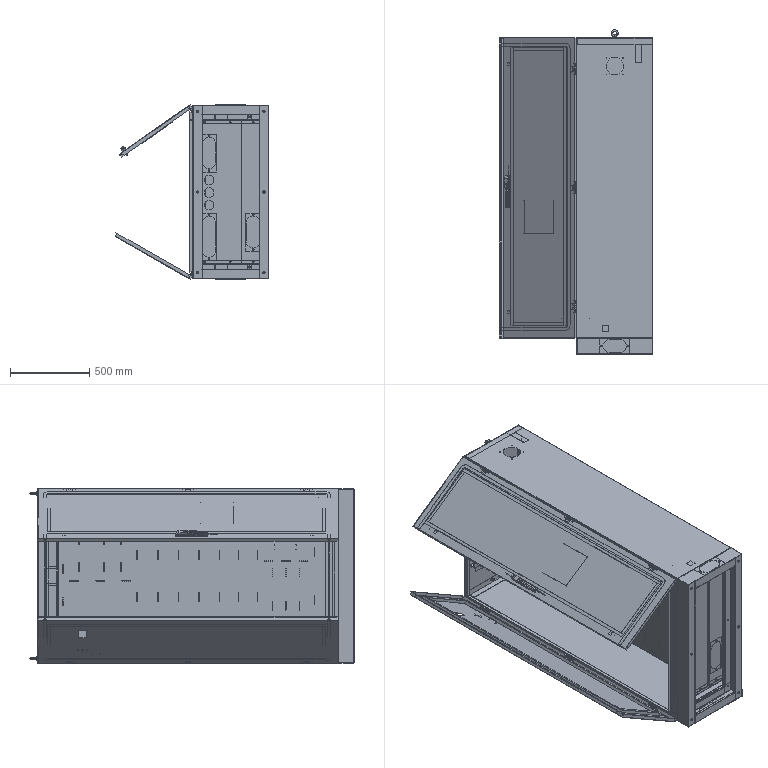Assembly | SolidWorks | mm | 69 component files | 71 solids | 3708 faces | box 971.82 x 2050.25 x 1105.32 mm | volume 17695028 mm3 | cylinder 1882 | plane 1722 | spline 100 | cone 4 | commonest cylinder face diameters 5 x728 7 x132 0.5 x108 0.2 x99 6 x92 3 x90 4 x86 8 x80
Bill of materials:
201LargeHinge | 6 |  | Elongated bracket with a hollow, open-sided box-section beam along one edge and a teardrop-profile side web ending in a cylindrical knuckle with a through bore; two knuckle segments are separated by a central gap, and internal cylindrical bosses with holes sit inside the beam.
BaseCableHoleBlankingPlate | 4 |  | Thin flat rectangular plate with two small round holes centered near its two short ends.
BottomFrameFront | 1 |  | Long, slender sheet-metal channel with a C-shaped cross-section, small-radius bends and short inward return lips; small holes are spaced along the length.
BottomFrameLeftAndRight | 2 |  | Sheet-metal cover/plate with a flat top panel, two bent-down side walls ending in short inward feet, flat end tabs extending past the walls, and a central obround cutout flanked by two small holes.
BottomFrameRear | 1 |  | Long sheet-metal channel with a C-shaped cross-section and short return lips; the web has two obround cutouts, each with small holes above and below it, plus small holes along the flanges and a small internal boss.
BottomBlankingPlateCableHoleBlankingPlate1 | 1 |  | Thin flat rectangular plate, narrower than tall, with two small round holes on the centerline near the short ends.
BottomBlankingPlateCableHoleBlankingPlate2 | 2 |  | Thin flat rectangular plate with two small round holes on the centerline near each short end.
BottomPlateMountingPlate1 | 1 |  | Flat rectangular sheet panel with very short bent edge flanges on the long sides; it has two large obround cutouts, three circular holes between them, small holes beside each cutout and small holes near the corners.
BottomPlateMountingPlate2 | 1 |  | Long, narrow flat sheet panel with short bent side flanges, a single obround cutout in the lower portion with small holes above and below it, and small holes near both ends.
ConnectingAngleIron | 1 |  | Thin L-shaped angle with roughly equal legs and a small inside bend radius; one leg is shorter in length than the other, which creates a step at one end.
ConnectingAngleIronSymmetric | 1 |  | Thin L-shaped angle with a small bend radius; the two legs differ in length, giving a step at one end. It appears to be a mirrored or reoriented version of a similar angle.
FrontLowerBeam | 1 |  | Long, slender sheet-metal profile with an asymmetric section: a top flange extending one way, a tall web, a bottom flange extending the other way and a short upturned lip; small holes are spaced along its length.
LeftSidePanel | 1 |  | Long, shallow rectangular tray made of thin plate. It has a flat base, low upturned flanges along both long edges and short turned-down end lips.
LimitSwitchBracket | 1 |  | Short equal-leg angle bracket with a rounded inside bend and two round through-holes in one leg.
MountingBeam | 1 |  | Long, slender angle profile with a rounded bend and one small hole near each end of one leg.
MountingPlateBracket | 2 |  | Square-legged L-bracket of thin plate with a round hole in the upright leg and a short cylindrical boss or sleeve on that leg.
RearDoorFixingPlate | 2 |  | Flat rectangular plate with two rounded corners along one edge and a large central round through-hole, similar to a square washer or tab.
RearLowerBeam | 1 |  | Long thin-walled formed profile with several bends, in a stepped open-channel shape. It has one small hole near mid-length and stepped or notched ends.
RightSidePlate | 1 |  | Long rectangular panel or cover with turned-down edges, one large round hole near one end and small holes around that hole.
ShelfSupportBeamLeft | 1 |  | Long stepped bracket rail with a Z- or hat-like section. It carries three evenly spaced cylindrical studs or bosses on one flange and a block-and-cylinder feature on another web.
ShelfSupportBeamRight | 1 |  | Long stepped bracket rail with a multi-bend profile, mirrored compared with unnamed part. It has three evenly spaced cylindrical studs or bosses.
TopCover | 1 |  | Rectangular sheet panel with stepped or offset flanges along its long edges. It has an obround slot near one end, small holes on either side of the slot, and small holes at the end centrelines.
TopLightBracket | 1 |  | Long C-channel with a flat web, short return flanges at each end of the section and two small holes in the web.
TopReinforcementAngleIron | 2 |  | Long equal-leg angle with one round hole at mid-length in the upright leg and a hex-shaped boss, likely a nut-like feature, on the inside face at that hole.
Triangle | 2 |  | Thin flat plate in the shape of a right triangle, with one circular through-hole near the right-angle corner.
CL201-1Hinge(ClawTypeAttachment) | 6 |  | Flat rectangular sheet leaf with one edge rolled into a hollow cylindrical barrel. The barrel is split into three knuckle segments separated by two gaps. It looks like a hinge leaf.
FrontDoorFlange | 1 |  | Long rectangular thin sheet panel with shallow turned-up or bent edges along the long sides and small notches near the ends. Near one end it has one small rectangular cutout and one small hole with small marks around it.
1760RectangularTube | 4 |  | Thin square frame made of slender bar stock with an open center. It looks like a closed square loop.
390RectangularTube | 4 |  | Straight bar with a square cross-section and flat square ends.
WireRack | 1 |  | Bent sheet strap: a flat rectangular web with a short leg bent down about 90 degrees at each end, forming a shallow U or cap profile with rounded bends.
DocumentBox | 1 |  | Rectangular flat plate or block with a V-shaped notch cut in from one edge. The notch ends in a rounded root.
FrontDoorLockHole | 1 |  | Long thin rectangular sheet panel with narrow bent edges along the long sides, small notches near the ends, and a few small slots or holes near one long edge.
LockRodBracket | 2 |  | L-shaped bent sheet bracket. One leg is a flat rectangle. The other leg, bent about 90 degrees, has a rounded end and a large circular through-hole.
LowerLockRod | 1 |  | Long slender round rod with a short jog (double bend) near one end and a pointed or chamfered tip at that end. The other end is a flattened section with two small holes.
M12LiftingEye | 2 |  | Eye-bolt-like part: a round ring (torus) joined to a cylindrical collar, with a smaller-diameter cylindrical shank extending from the collar.
MountingPlate | 1 |  | Long narrow sheet channel with a shallow U cross-section and rounded corners. There is one small elongated hole near each end of the web.
MS830ConnectingRodLock | 1 |  | Long, narrow multi-piece-looking body: a stepped, box-like housing with a chamfered upper end, sitting on a flat strip. The strip runs past both ends as flat tabs, each with two round holes, and is joggled (offset) where it leaves the housing. A small round knob or disc with a slot sits on one side face, near a rectangular block.
RearDoorPanel | 1 |  | Thin, flat rectangular plate, about twice as long as it is tall, with uniform thickness and no clear cutouts.
RearDoorStiffener | 1 |  | Long, straight, thin-walled formed profile of constant cross-section. The end view shows a hat (top-hat) shape: a central web, two legs turning toward the same side, and short lips at the ends of the legs turning away from each other.
Shelf | 1 |  | Thin, flat rectangular plate with many small perforations in short straight rows, mostly vertical with some horizontal, spread across the face in a grid-like layout.
TopCoverCableHoleBlankingPlate | 1 |  | Thin, flat rectangular plate, about twice as long as it is tall, with one round through-hole near each short end, both at mid-height.
UpperLockRod | 1 |  | Long, slender round rod. Near one end it has a short joggle (an offset bend in two steps), ending in a short straight tip. The other end is a short flattened or rectangular section with two small holes.
Mates:
1. coincident | CabinetWelding-1/FrontLowerBeam-1 face at (108.182, -1006.927, 1410.006) dir (0, -1, 0) | BaseWeldment-1/BottomFrameLeftAndRight-1 face at (-18040.001, -1006.927, 9206.843) dir (0, 1, 0)
2. coincident | CabinetWelding-1/RightSidePlate-1 face at (-10032.487, -6118.242, 2450.006) dir (0, 0, 1) | BaseWeldment-1/BottomFrameLeftAndRight-1 face at (-18040.001, -7766.065, 2450.006) dir (0, 0, 1)
3. coincident | CabinetWelding-1/FrontLowerBeam-1 face at (107.082, -1006.227, 1410.006) dir (-1, 0, 0) | BaseWeldment-1/BottomFrameFront-1 face at (107.082, -7813.138, -16268.116) dir (-1, 0, 0)
4. coincident | BaseWeldment-1/BottomFrameRear-1 face at (587.082, -6857.662, 20235.861) dir (1, 0, 0) | BaseCableHoleBlankingPlate-1 face at (587.082, -8620.302, -16132.916) dir (-1, 0, 0)
5. concentric | BaseWeldment-1/BottomFrameRear-1 face at (585.582, -1056.927, 2115.006) dir (1, 0, 0) r 4 | BaseCableHoleBlankingPlate-1 face at (587.982, -1056.927, 2115.006) dir (-1, 0, 0) r 3.5
6. concentric | BaseWeldment-1/BottomFrameRear-1 face at (585.582, -1056.927, 2285.006) dir (1, 0, 0) r 4 | BaseCableHoleBlankingPlate-1 face at (587.982, -1056.927, 2285.006) dir (-1, 0, 0) r 3.5
7. coincident | BaseWeldment-1/BottomFrameRear-1 face at (587.082, -6857.662, 20235.861) dir (1, 0, 0) | BaseCableHoleBlankingPlate-2 face at (587.082, -8620.302, -16732.916) dir (-1, 0, 0)
8. concentric | BaseWeldment-1/BottomFrameRear-1 face at (585.582, -1056.927, 1515.006) dir (1, 0, 0) r 4 | BaseCableHoleBlankingPlate-2 face at (587.982, -1056.927, 1515.006) dir (-1, 0, 0) r 3.5
9. concentric | BaseWeldment-1/BottomFrameRear-1 face at (585.582, -1056.927, 1685.006) dir (1, 0, 0) r 4 | BaseCableHoleBlankingPlate-2 face at (587.982, -1056.927, 1685.006) dir (-1, 0, 0) r 3.5
10. coincident | BaseWeldment-1/BottomFrameLeftAndRight-2 face at (18734.165, -7766.065, 1350.006) dir (0, 0, -1) | BaseCableHoleBlankingPlate-3 face at (-17985.84, -8620.302, 1350.006) dir (0, 0, 1)
11. concentric | BaseWeldment-1/BottomFrameLeftAndRight-2 face at (432.082, -1056.927, 1351.506) dir (0, 0, -1) r 4 | BaseCableHoleBlankingPlate-3 face at (432.082, -1056.927, 1349.106) dir (0, 0, 1) r 3.5
12. concentric | BaseWeldment-1/BottomFrameLeftAndRight-2 face at (262.082, -1056.927, 1351.506) dir (0, 0, -1) r 4 | BaseCableHoleBlankingPlate-3 face at (262.082, -1056.927, 1349.106) dir (0, 0, 1) r 3.5
13. coincident | BaseWeldment-1/BottomFrameLeftAndRight-1 face at (-18040.001, -7766.065, 2450.006) dir (0, 0, 1) | BaseCableHoleBlankingPlate-4 face at (-17985.84, -8620.302, 2450.006) dir (0, 0, -1)
14. concentric | BaseWeldment-1/BottomFrameLeftAndRight-1 face at (432.082, -1056.927, 2448.506) dir (0, 0, 1) r 4 | BaseCableHoleBlankingPlate-4 face at (432.082, -1056.927, 2450.006) dir (0, 0, 1) r 3.5
15. concentric | BaseWeldment-1/BottomFrameLeftAndRight-1 face at (262.082, -1056.927, 2448.506) dir (0, 0, 1) r 4 | BaseCableHoleBlankingPlate-4 face at (262.082, -1056.927, 2450.006) dir (0, 0, 1) r 3.5
16. coincident | CabinetWelding-1/TopCover-1 face at (-6180.575, 893.073, -11058.588) dir (0, 1, 0) | TopCoverCableHoleBlankingPlate-1 face at (-18406.867, 893.073, 8560.424) dir (0, -1, 0)
17. concentric | CabinetWelding-1/TopCover-1 face at (217.082, 891.873, 1571.206) dir (0, 1, 0) r 4 | TopCoverCableHoleBlankingPlate-1 face at (217.082, 893.073, 1571.206) dir (0, 1, 0) r 3.5
18. concentric | CabinetWelding-1/TopCover-1 face at (477.082, 891.873, 1571.206) dir (0, 1, 0) r 4 | TopCoverCableHoleBlankingPlate-1 face at (477.082, 893.073, 1571.206) dir (0, 1, 0) r 3.5
19. coincident | CabinetWelding-1/ShelfSupportBeamLeft-1 face at (-23700.714, -948.127, 8695.02) dir (0, 1, 0) | Shelf-1 face at (6604.247, -948.127, -24609.222) dir (0, -1, 0)
20. concentric | CabinetWelding-1/ShelfSupportBeamLeft-1 face at (466.182, -949.927, 1425.006) dir (0, 1, 0) r 4 | Shelf-1 face at (466.182, -946.327, 1425.006) dir (0, -1, 0) r 4
21. parallel | CabinetWelding-1/FrontLowerBeam-1 face at (107.082, -1006.227, 1410.006) dir (-1, 0, 0) | Shelf-1 face at (451.982, -7097.393, -24609.222) dir (-1, 0, 0)
22. coincident | CabinetWelding-1/ShelfSupportBeamLeft-1 face at (-23700.714, -971.327, 8674.22) dir (0, 1, 0) | BottomPlateMountingPlate1-1 face at (-6898.53, -971.327, -27327.264) dir (0, -1, 0)
23. distance | BottomPlateMountingPlate1-1 face at (413.382, -971.327, 2353.506) dir (0, 0, 1) | CabinetWelding-1/ShelfSupportBeamRight-1 face at (-23700.714, -8201.141, 2355.006) dir (0, 0, -1)
24. distance | BottomPlateMountingPlate1-1 face at (109.382, -7979.84, -27327.264) dir (-1, 0, 0) | BaseWeldment-1/BottomFrameFront-1 face at (107.082, -7813.138, -16268.116) dir (-1, 0, 0)
25. coincident | CabinetWelding-1/ShelfSupportBeamLeft-1 face at (-23700.714, -971.327, 8674.22) dir (0, 1, 0) | BottomPlateMountingPlate2-1 face at (-6353.567, -971.327, -29538.735) dir (0, -1, 0)
26. coincident | BottomPlateMountingPlate1-1 edge at (413.382, -970.127, 1446.506) dir (-1, 0, 0) | BottomPlateMountingPlate2-1 face at (413.882, -971.327, 1446.506) dir (0, 0, -1)
27. distance | BottomPlateMountingPlate2-1 face at (563.882, 5945.522, -29538.735) dir (1, 0, 0) | CabinetWelding-1/RearLowerBeam-1 face at (587.082, -6464.106, 7747.219) dir (1, 0, 0)
28. coincident | BottomPlateMountingPlate1-1 face at (-6898.53, -970.127, -27327.264) dir (0, 1, 0) | BottomBlankingPlateCableHoleBlankingPlate1-1 face at (-6643.041, -970.127, -32139.241) dir (0, -1, 0)
29. concentric | BottomPlateMountingPlate1-1 face at (210.382, -971.327, 1476.506) dir (0, 1, 0) r 4 | BottomBlankingPlateCableHoleBlankingPlate1-1 face at (210.382, -970.127, 1476.506) dir (0, 1, 0) r 3.5
30. concentric | BottomPlateMountingPlate1-1 face at (210.382, -971.327, 1756.506) dir (0, 1, 0) r 4 | BottomBlankingPlateCableHoleBlankingPlate1-1 face at (210.382, -970.127, 1756.506) dir (0, 1, 0) r 3.5
31. coincident | BottomPlateMountingPlate1-1 face at (-6898.53, -970.127, -27327.264) dir (0, 1, 0) | BottomBlankingPlateCableHoleBlankingPlate2-1 face at (7392.9, -970.127, -31716.912) dir (0, -1, 0)
32. concentric | BottomPlateMountingPlate1-1 face at (210.382, -971.327, 2256.506) dir (0, 1, 0) r 4 | BottomBlankingPlateCableHoleBlankingPlate2-1 face at (210.382, -969.127, 2256.506) dir (0, -1, 0) r 3.5
33. concentric | BottomPlateMountingPlate1-1 face at (210.382, -971.327, 2036.506) dir (0, 1, 0) r 4 | BottomBlankingPlateCableHoleBlankingPlate2-1 face at (210.382, -969.127, 2036.506) dir (0, -1, 0) r 3.5
34. coincident | BottomPlateMountingPlate2-1 face at (-6353.567, -970.127, -29538.735) dir (0, 1, 0) | BottomBlankingPlateCableHoleBlankingPlate2-2 face at (7671.4, -970.127, -32216.912) dir (0, -1, 0)
35. concentric | BottomPlateMountingPlate2-1 face at (488.882, -971.327, 1756.506) dir (0, 1, 0) r 4 | BottomBlankingPlateCableHoleBlankingPlate2-2 face at (488.882, -969.127, 1756.506) dir (0, -1, 0) r 3.5
36. concentric | BottomPlateMountingPlate2-1 face at (488.882, -971.327, 1536.506) dir (0, 1, 0) r 4 | BottomBlankingPlateCableHoleBlankingPlate2-2 face at (488.882, -969.127, 1536.506) dir (0, -1, 0) r 3.5
37. coincident | CabinetWelding-1/LeftSidePanel-1 face at (587.082, -6066.431, 8611.136) dir (1, 0, 0) | RearDoorPanelWeldment-1/RearDoorPanel-1 face at (587.082, -6903.085, 22902.405) dir (1, 0, 0)
38. distance | RearDoorPanelWeldment-1/RearDoorPanel-1 face at (-5372.376, -945.427, 22902.405) dir (0, -1, 0) | CabinetWelding-1/RearLowerBeam-1 face at (6102.461, -946.927, 7747.219) dir (0, 1, 0)
39. distance | RearDoorPanelWeldment-1/RearDoorPanel-1 face at (-19913.917, -6903.085, 2403.206) dir (0, 0, 1) | CabinetWelding-1/RightSidePlate-1 face at (11248.051, -6118.242, 2405.006) dir (0, 0, -1)
40. coincident | CabinetWelding-1/MountingPlateBracket-1 face at (287.77, -926.927, 1354.662) dir (0, 1, 0) | MountingPlate-1 face at (8130.269, -926.927, -33580.048) dir (0, -1, 0)
41. distance | MountingPlate-1 face at (345.532, -925.427, 1357.506) dir (0, 0, -1) | CabinetWelding-1/LeftSidePanel-1 face at (7846.412, -6066.431, 1350.006) dir (0, 0, -1)
42. distance | MountingPlate-1 face at (246.332, 6956.21, -33580.048) dir (-1, 0, 0) | CabinetWelding-1/MountingPlateBracket-1 face at (267.082, -928.427, 1391.206) dir (-1, 0, 0)
43. parallel | CabinetWelding-1/LeftSidePanel-1 face at (107.082, -6066.431, -6387.524) dir (-1, 0, 0) | 201LargeHinge-2 face at (107.082, 657.073, 1372.506) dir (1, 0, 0)
44. coincident | CabinetWelding-1/LeftSidePanel-1 face at (107.082, -6066.431, -6387.524) dir (-1, 0, 0) | 201LargeHinge-2 face at (107.082, 657.073, 1372.506) dir (1, 0, 0)
45. concentric | CabinetWelding-1/LeftSidePanel-1 face at (117.082, 719.073, 1378.006) dir (-1, 0, 0) r 3.5 | 201LargeHinge-2 face at (94.082, 719.073, 1378.006) dir (1, 0, 0) r 3
46. concentric | CabinetWelding-1/LeftSidePanel-1 face at (117.082, 669.073, 1378.006) dir (-1, 0, 0) r 3.5 | 201LargeHinge-2 face at (94.082, 669.073, 1378.006) dir (1, 0, 0) r 3
47. concentric | CabinetWelding-1/LeftSidePanel-1 face at (117.082, -80.927, 1378.006) dir (-1, 0, 0) r 3.5 | 201LargeHinge-3 face at (94.082, -80.927, 1378.006) dir (1, 0, 0) r 3
48. concentric | CabinetWelding-1/LeftSidePanel-1 face at (117.082, -30.927, 1378.006) dir (-1, 0, 0) r 3.5 | 201LargeHinge-3 face at (94.082, -30.927, 1378.006) dir (1, 0, 0) r 3
49. coincident | CabinetWelding-1/LeftSidePanel-1 face at (107.082, -6066.431, -6387.524) dir (-1, 0, 0) | 201LargeHinge-3 face at (107.082, -92.927, 1372.506) dir (1, 0, 0)
50. concentric | CabinetWelding-1/LeftSidePanel-1 face at (117.082, -830.927, 1378.006) dir (-1, 0, 0) r 3.5 | 201LargeHinge-4 face at (94.082, -830.927, 1378.006) dir (1, 0, 0) r 3
51. concentric | CabinetWelding-1/LeftSidePanel-1 face at (117.082, -780.927, 1378.006) dir (-1, 0, 0) r 3.5 | 201LargeHinge-4 face at (94.082, -780.927, 1378.006) dir (1, 0, 0) r 3
52. coincident | CabinetWelding-1/LeftSidePanel-1 face at (107.082, -6066.431, -6387.524) dir (-1, 0, 0) | 201LargeHinge-4 face at (107.082, -842.927, 1372.506) dir (1, 0, 0)
53. concentric | CabinetWelding-1/RightSidePlate-1 face at (117.082, 719.073, 2422.006) dir (-1, 0, 0) r 3.5 | 201LargeHinge-5 face at (94.082, 719.073, 2422.006) dir (1, 0, 0) r 3
54. concentric | CabinetWelding-1/RightSidePlate-1 face at (117.082, 669.073, 2422.006) dir (-1, 0, 0) r 3.5 | 201LargeHinge-5 face at (94.082, 669.073, 2422.006) dir (1, 0, 0) r 3
55. coincident | CabinetWelding-1/RightSidePlate-1 face at (107.082, -6118.242, -7691.363) dir (-1, 0, 0) | 201LargeHinge-5 face at (107.082, 731.073, 2427.506) dir (1, 0, 0)
56. concentric | CabinetWelding-1/RightSidePlate-1 face at (117.082, -30.927, 2422.006) dir (-1, 0, 0) r 3.5 | 201LargeHinge-6 face at (94.082, -30.927, 2422.006) dir (1, 0, 0) r 3
57. concentric | CabinetWelding-1/RightSidePlate-1 face at (117.082, -80.927, 2422.006) dir (-1, 0, 0) r 3.5 | 201LargeHinge-6 face at (94.082, -80.927, 2422.006) dir (1, 0, 0) r 3
58. coincident | CabinetWelding-1/RightSidePlate-1 face at (107.082, -6118.242, -7691.363) dir (-1, 0, 0) | 201LargeHinge-6 face at (107.082, -18.927, 2427.506) dir (1, 0, 0)
59. concentric | CabinetWelding-1/RightSidePlate-1 face at (117.082, -780.927, 2422.006) dir (-1, 0, 0) r 3.5 | 201LargeHinge-7 face at (94.082, -780.927, 2422.006) dir (1, 0, 0) r 3
60. concentric | CabinetWelding-1/RightSidePlate-1 face at (117.082, -830.927, 2422.006) dir (-1, 0, 0) r 3.5 | 201LargeHinge-7 face at (94.082, -830.927, 2422.006) dir (1, 0, 0) r 3
61. coincident | CabinetWelding-1/RightSidePlate-1 face at (107.082, -6118.242, -7691.363) dir (-1, 0, 0) | 201LargeHinge-7 face at (107.082, -768.927, 2427.506) dir (1, 0, 0)
62. concentric | 201LargeHinge-5 face at (90.082, 731.073, 2442.506) dir (0, -1, 0) r 3.5 | FrontDoorLockHoleWeld-2/CL201-1Hinge(ClawTypeAttachment)-1 face at (90.082, 676.073, 2442.506) dir (0, 1, 0) r 3.5
63. coincident | 201LargeHinge-5 face at (107.082, 676.073, 2450.661) dir (0, 1, 0) | FrontDoorLockHoleWeld-2/CL201-1Hinge(ClawTypeAttachment)-1 face at (87.557, 676.073, 2437.063) dir (0, -1, 0)
64. concentric | 201LargeHinge-2 face at (90.082, 657.073, 1357.506) dir (0, 1, 0) r 3.5 | FrontDoorFlangeWelding-2/CL201-1Hinge(ClawTypeAttachment)-1 face at (90.082, 710.073, 1357.506) dir (0, -1, 0) r 3.5
65. coincident | 201LargeHinge-2 face at (107.082, 676.073, 1349.351) dir (0, 1, 0) | FrontDoorFlangeWelding-2/CL201-1Hinge(ClawTypeAttachment)-1 face at (88.322, 676.073, 1360.531) dir (0, -1, 0)
66. coincident | FrontDoorLockHoleWeld-2/FrontDoorLockHole-1 face at (-326.791, -36.427, 2146.97) dir (0.818, 0, 0.5751) | MS830ConnectingRodLock-1 face at (-332.543, -36.427, 2155.15) dir (-0.818, 0, -0.5751)
67. coincident | FrontDoorLockHoleWeld-2/FrontDoorLockHole-1 face at (-315.747, -36.427, 2154.734) dir (0, -1, 0) | MS830ConnectingRodLock-1 face at (-317.409, -36.427, 2165.79) dir (0, 1, 0)
68. coincident | FrontDoorLockHoleWeld-2/FrontDoorLockHole-1 face at (-335.696, 817.607, 2152.933) dir (-0.5751, 0, 0.818) | MS830ConnectingRodLock-1 face at (-310.864, 20.573, 2170.392) dir (0.5751, 0, -0.818)
69. coincident | MS830ConnectingRodLock-1 face at (-323.902, 30.073, 2156.335) dir (0.818, 0, 0.5751) | UpperLockRod-1 face at (-322.156, 100.073, 2153.852) dir (-0.818, 0, -0.5751)
70. concentric | MS830ConnectingRodLock-1 face at (-319.755, 75.073, 2151.306) dir (-0.818, 0, -0.5751) r 3 | UpperLockRod-1 face at (-365.974, 75.073, 2118.81) dir (0.818, 0, 0.5751) r 2.1
71. concentric | MS830ConnectingRodLock-1 face at (-319.755, 50.073, 2151.306) dir (-0.818, 0, -0.5751) r 3 | UpperLockRod-1 face at (-365.974, 50.073, 2118.81) dir (0.818, 0, 0.5751) r 2.1
72. coincident | MS830ConnectingRodLock-1 face at (-321.448, -188.927, 2158.061) dir (-0.818, 0, -0.5751) | LowerLockRod-1 face at (-319.702, -259.927, 2155.577) dir (0.818, 0, 0.5751)
73. concentric | MS830ConnectingRodLock-1 face at (-315.255, -209.927, 2154.469) dir (-0.818, 0, -0.5751) r 3 | LowerLockRod-1 face at (-271.899, -209.927, 2184.952) dir (-0.818, 0, -0.5751) r 2.1
74. concentric | MS830ConnectingRodLock-1 face at (-315.255, -234.927, 2154.469) dir (-0.818, 0, -0.5751) r 3 | LowerLockRod-1 face at (-271.899, -234.927, 2184.952) dir (-0.818, 0, -0.5751) r 2.1
75. concentric | CabinetWelding-1/TopReinforcementAngleIron-1 face at (347.082, 879.873, 1378.206) dir (0, 1, 0) r 6 | M12LiftingEye-1 face at (347.082, 873.073, 1378.206) dir (0, 1, 0) r 6
76. coincident | CabinetWelding-1/TopCover-1 face at (-6180.575, 893.073, -11058.588) dir (0, 1, 0) | M12LiftingEye-1 face at (347.082, 893.073, 1377.729) dir (0, -1, 0)
77. concentric | CabinetWelding-1/TopReinforcementAngleIron-2 face at (347.082, 414.873, 2421.806) dir (0, 1, 0) r 7 | M12LiftingEye-2 face at (347.082, 873.073, 2421.806) dir (0, 1, 0) r 6
78. coincident | CabinetWelding-1/TopCover-1 face at (-6180.575, 893.073, -11058.588) dir (0, 1, 0) | M12LiftingEye-2 face at (347.082, 893.073, 2421.329) dir (0, -1, 0)
79. coincident | BottomFrameFront-1 face at (-17977.695, -76.18, 7933.912) dir (0, 1, 0) | BottomFrameLeftAndRight-1 face at (7497.264, -76.18, 19277.085) dir (0, 1, 0)
80. coincident | BottomFrameFront-1 face at (-17977.695, 6785.43, 1070.002) dir (0, 0, -1) | BottomFrameLeftAndRight-1 face at (739.627, -77.68, 1070.002) dir (0, 0, 1)
81. coincident | BottomFrameRear-1 face at (18526.282, -76.18, -5198.433) dir (0, 1, 0) | BottomFrameLeftAndRight-1 face at (7497.264, -76.18, 19277.085) dir (0, 1, 0)
82. coincident | BottomFrameRear-1 face at (18526.282, 5829.955, 710.002) dir (0, 0, 1) | BottomFrameLeftAndRight-1 face at (681.927, -88.18, 710.002) dir (0, 0, -1)
83. coincident | BottomFrameFront-1 face at (-17977.695, -76.18, 7933.912) dir (0, 1, 0) | BottomFrameLeftAndRight-2 face at (-7116.41, -76.18, -17497.081) dir (0, 1, 0)
84. coincident | BottomFrameRear-1 face at (18526.282, 5829.955, 710.002) dir (0, 0, 1) | BottomFrameLeftAndRight-2 face at (-358.773, -77.68, 710.002) dir (0, 0, -1)
85. coincident | BottomFrameRear-1 face at (740.427, -233.88, 651.502) dir (1, 0, 0) | BottomFrameLeftAndRight-1 face at (740.427, -6835.317, 19277.085) dir (1, 0, 0)
86. coincident | BottomFrameFront-1 face at (740.427, -18.48, 1128.502) dir (1, 0, 0) | BottomFrameLeftAndRight-1 face at (740.427, -6835.317, 19277.085) dir (1, 0, 0)
87. coincident | BottomFrameFront-1 face at (-359.573, -233.88, 1128.502) dir (-1, 0, 0) | BottomFrameLeftAndRight-2 face at (-359.573, -6835.317, -17497.081) dir (-1, 0, 0)
88. coincident | RightSidePlate-1 face at (501.453, -6278.113, 12552.171) dir (1, 0, 0) | RearLowerBeam-1 face at (501.453, -6623.978, 7231.614) dir (1, 0, 0)
89. coincident | RightSidePlate-1 face at (500.253, -1106.799, 1890.502) dir (0, 0, -1) | RearLowerBeam-1 face at (500.253, -1166.099, 1890.502) dir (0, 0, 1)
90. coincident | RightSidePlate-1 face at (-10118.116, -1166.799, -3178.713) dir (0, -1, 0) | RearLowerBeam-1 face at (-4957.525, -1166.799, 7231.614) dir (0, -1, 0)
91. coincident | LeftSidePanel-1 face at (501.453, -6226.303, 8095.532) dir (1, 0, 0) | RearLowerBeam-1 face at (501.453, -6623.978, 7231.614) dir (1, 0, 0)
92. coincident | LeftSidePanel-1 face at (7760.784, -1166.799, 5895.705) dir (0, -1, 0) | RearLowerBeam-1 face at (-4957.525, -1166.799, 7231.614) dir (0, -1, 0)
93. coincident | LeftSidePanel-1 face at (500.253, -1106.799, 878.302) dir (0, 0, 1) | RearLowerBeam-1 face at (500.253, -1063.399, 878.302) dir (0, 0, -1)
94. coincident | LeftSidePanel-1 face at (21.453, -6226.303, -6903.129) dir (-1, 0, 0) | FrontLowerBeam-1 face at (21.453, -1166.099, 894.402) dir (-1, 0, 0)
95. coincident | LeftSidePanel-1 face at (22.653, -1166.799, 878.302) dir (0, 0, 1) | FrontLowerBeam-1 face at (22.653, -1166.099, 878.302) dir (0, 0, -1)
96. coincident | LeftSidePanel-1 face at (7760.784, -1166.799, 5895.705) dir (0, -1, 0) | FrontLowerBeam-1 face at (22.553, -1166.799, 894.402) dir (0, -1, 0)
97. coincident | LeftSidePanel-1 face at (7760.784, -6226.303, 835.602) dir (0, 0, 1) | TopCover-1 face at (22.553, 732.001, 835.602) dir (0, 0, -1)
98. coincident | LeftSidePanel-1 face at (21.453, -6226.303, -6903.129) dir (-1, 0, 0) | TopCover-1 face at (21.453, -5556.257, -11574.193) dir (-1, 0, 0)
99. coincident | LeftSidePanel-1 face at (22.653, 733.201, 878.302) dir (0, 1, 0) | TopCover-1 face at (-6266.204, 733.201, -11574.193) dir (0, 1, 0)
100. coincident | RearLowerBeam-1 face at (500.253, -6623.978, 7231.614) dir (-1, 0, 0) | ShelfSupportBeamLeft-1 face at (500.253, -1109.799, 852.402) dir (1, 0, 0)
101. coincident | RightSidePlate-1 face at (500.253, -6278.113, 12552.171) dir (-1, 0, 0) | ShelfSupportBeamRight-1 face at (500.253, -1107.999, 1916.402) dir (1, 0, 0)
102. coincident | ShelfSupportBeamLeft-1 face at (-23786.342, -1107.999, 8179.415) dir (0, 1, 0) | ShelfSupportBeamRight-1 face at (-23786.342, -1107.999, -5410.612) dir (0, 1, 0)
103. distance | ShelfSupportBeamRight-1 face at (-23786.342, 6179.014, 1879.402) dir (0, 0, 1) | RightSidePlate-1 face at (-10118.116, -6278.113, 1934.402) dir (0, 0, 1)
104. distance | ShelfSupportBeamLeft-1 face at (-23786.342, 6179.014, 889.402) dir (0, 0, -1) | LeftSidePanel-1 face at (7760.784, -6226.303, 834.402) dir (0, 0, -1)
105. coincident | RearLowerBeam-1 face at (6016.832, -1107.999, 7231.614) dir (0, -1, 0) | ShelfSupportBeamLeft-1 face at (-23786.342, -1107.999, 8179.415) dir (0, 1, 0)
106. coincident | LeftSidePanel-1 face at (7760.784, -6226.303, 835.602) dir (0, 0, 1) | MountingPlateBracket-1 face at (202.141, -1086.799, 835.602) dir (0, 0, -1)
107. distance | MountingPlateBracket-1 face at (202.141, -1086.799, 839.057) dir (0, 1, 0) | FrontLowerBeam-1 face at (22.553, -1166.799, 894.402) dir (0, -1, 0)
108. distance | MountingPlateBracket-1 face at (181.453, -1126.799, 835.602) dir (-1, 0, 0) | LeftSidePanel-1 face at (21.453, -6226.303, -6903.129) dir (-1, 0, 0)
109. coincident | RightSidePlate-1 face at (-10118.116, -6278.113, 1933.202) dir (0, 0, -1) | MountingPlateBracket-2 face at (200.766, -1086.799, 1933.202) dir (0, 0, 1)
110. coincident | MountingPlateBracket-1 face at (202.141, -1086.799, 839.057) dir (0, 1, 0) | MountingPlateBracket-2 face at (200.766, -1086.799, 1929.746) dir (0, 1, 0)
111. coincident | MountingPlateBracket-1 face at (181.453, -1126.799, 835.602) dir (-1, 0, 0) | MountingPlateBracket-2 face at (181.453, -1088.299, 1933.202) dir (-1, 0, 0)
112. coincident | TopCover-1 face at (-6266.204, 732.001, -11574.193) dir (0, -1, 0) | TopLightBracket-1 face at (101.453, 732.001, 1704.402) dir (0, 1, 0)
113. distance | TopLightBracket-1 face at (61.453, 687.001, 1653.409) dir (-1, 0, 0) | TopCover-1 face at (21.453, -5556.257, -11574.193) dir (-1, 0, 0)
114. distance | TopLightBracket-1 face at (58.466, 687.001, 1704.402) dir (0, 0, 1) | RightSidePlate-1 face at (-10118.116, -6278.113, 1934.402) dir (0, 0, 1)
115. coincident | TopCover-1 face at (-6223.604, 688.201, -11574.193) dir (0, -1, 0) | LimitSwitchBracket-1 face at (-7469.264, 688.201, -37543.327) dir (0, -1, 0)
116. coincident | TopCover-1 face at (22.653, -5556.257, -11574.193) dir (1, 0, 0) | LimitSwitchBracket-1 face at (22.653, 8181.719, -37543.327) dir (-1, 0, 0)
117. distance | LimitSwitchBracket-1 face at (42.653, 688.201, 1866.402) dir (0, 0, 1) | RightSidePlate-1 face at (-10118.116, -6278.113, 1934.402) dir (0, 0, 1)
118. coincident | LeftSidePanel-1 face at (7760.784, -6226.303, 835.602) dir (0, 0, 1) | TopReinforcementAngleIron-1 face at (24.453, 732.001, 835.602) dir (0, 0, -1)
119. coincident | TopCover-1 face at (-6266.204, 732.001, -11574.193) dir (0, -1, 0) | TopReinforcementAngleIron-1 face at (24.453, 732.001, 835.602) dir (0, 1, 0)
120. distance | TopReinforcementAngleIron-1 face at (24.453, 670.796, 870.363) dir (-1, 0, 0) | LeftSidePanel-1 face at (21.453, -6226.303, -6903.129) dir (-1, 0, 0)
121. coincident | RightSidePlate-1 face at (-10118.116, -6278.113, 1933.202) dir (0, 0, -1) | TopReinforcementAngleIron-2 face at (498.453, 732.001, 1933.202) dir (0, 0, 1)
122. coincident | TopCover-1 face at (-6266.204, 732.001, -11574.193) dir (0, -1, 0) | TopReinforcementAngleIron-2 face at (498.453, 732.001, 1933.202) dir (0, 1, 0)
123. distance | TopReinforcementAngleIron-2 face at (24.453, 670.796, 1898.44) dir (-1, 0, 0) | RightSidePlate-1 face at (21.453, -6278.113, -8206.968) dir (-1, 0, 0)
124. coincident | TopReinforcementAngleIron-1 face at (24.453, 729.001, 838.602) dir (0, -1, 0) | ConnectingAngleIron-1 face at (392.353, 729.001, 835.602) dir (0, 1, 0)
125. distance | ConnectingAngleIron-1 face at (390.553, 669.43, 859.667) dir (-1, 0, 0) | LeftSidePanel-1 face at (501.453, -6226.303, 8095.532) dir (1, 0, 0)
126. coincident | LeftSidePanel-1 face at (7760.784, -6226.303, 835.602) dir (0, 0, 1) | ConnectingAngleIron-1 face at (390.553, 669.43, 835.602) dir (0, 0, -1)
127. coincident | RightSidePlate-1 face at (-10118.116, -6278.113, 1933.202) dir (0, 0, -1) | ConnectingAngleIronSymmetric-1 face at (392.353, 669.43, 1933.202) dir (0, 0, 1)
128. coincident | TopReinforcementAngleIron-2 face at (498.453, 729.001, 1930.202) dir (0, -1, 0) | ConnectingAngleIronSymmetric-1 face at (390.553, 729.001, 1933.202) dir (0, 1, 0)
129. coincident | ConnectingAngleIron-1 face at (390.553, 669.43, 859.667) dir (-1, 0, 0) | ConnectingAngleIronSymmetric-1 face at (390.553, 669.43, 1909.136) dir (-1, 0, 0)
130. coincident | ConnectingAngleIron-1 face at (392.353, 669.43, 859.667) dir (1, 0, 0) | MountingBeam-2 face at (392.353, 571.578, 892.297) dir (-1, 0, 0)
131. coincident | ConnectingAngleIron-1 face at (430.553, 574.001, 835.602) dir (0, -1, 0) | MountingBeam-2 face at (395.353, 574.001, 839.402) dir (0, -1, 0)
132. distance | MountingBeam-2 face at (395.353, 614.001, 1929.402) dir (0, 0, 1) | RightSidePlate-1 face at (-10118.116, -6278.113, 1934.402) dir (0, 0, 1)
133. coincident | TopCover-1 face at (480.653, 7518.658, -11574.193) dir (1, 0, 0) | Triangle-1 face at (480.653, 614.451, 1878.397) dir (1, 0, 0)
134. coincident | RightSidePlate-1 face at (479.453, 688.201, 1865.602) dir (0, 0, -1) | Triangle-1 face at (480.653, 664.401, 1865.602) dir (0, 0, 1)
135. coincident | TopCover-1 face at (479.453, 664.401, 903.402) dir (0, -1, 0) | Triangle-1 face at (480.653, 664.401, 1825.602) dir (0, 1, 0)
136. coincident | LeftSidePanel-1 face at (480.653, -6226.303, 8075.932) dir (1, 0, 0) | Triangle-2 face at (480.653, 677.196, 953.151) dir (1, 0, 0)
137. coincident | LeftSidePanel-1 face at (479.453, 688.201, 903.202) dir (0, 0, 1) | Triangle-2 face at (480.653, 624.401, 903.202) dir (0, 0, -1)
138. coincident | TopCover-1 edge at (480.653, 664.401, 1865.602) dir (0, 0, -1) | Triangle-2 face at (480.653, 664.401, 903.202) dir (0, 1, 0)
139. coincident | LeftSidePanel-1 face at (480.653, -6226.303, 8075.932) dir (1, 0, 0) | RearDoorFixingPlate-1 face at (480.653, -216.299, 915.202) dir (1, 0, 0)
140. coincident | LeftSidePanel-1 face at (470.653, -219.299, 905.955) dir (0, 1, 0) | RearDoorFixingPlate-1 face at (480.653, -219.299, 898.202) dir (0, -1, 0)
141. coincident | LeftSidePanel-1 face at (470.653, -199.299, 898.202) dir (0, 0, 1) | RearDoorFixingPlate-1 face at (480.653, -199.299, 898.202) dir (0, 0, -1)
142. coincident | RightSidePlate-1 face at (480.653, -6278.113, 12571.771) dir (1, 0, 0) | RearDoorFixingPlate-2 face at (480.653, -216.299, 1853.602) dir (1, 0, 0)
143. coincident | RightSidePlate-1 face at (470.653, -199.299, 1870.602) dir (0, 0, -1) | RearDoorFixingPlate-2 face at (479.453, -199.299, 1870.602) dir (0, 0, 1)
144. coincident | RightSidePlate-1 face at (470.653, -199.299, 1863.034) dir (0, -1, 0) | RearDoorFixingPlate-2 face at (479.453, -199.299, 1870.602) dir (0, 1, 0)
145. coincident | FrontDoorFlange-1 face at (-121.287, 1030.147, 1910) dir (0, 0, -1) | CL201-1Hinge(ClawTypeAttachment)-1 face at (-118.933, 922.613, 1910) dir (0, 0, 1)
146. distance | CL201-1Hinge(ClawTypeAttachment)-1 face at (-118.933, 922.613, 1907.5) dir (1, 0, 0) | FrontDoorFlange-1 face at (-147.433, 1030.147, 1911.5) dir (-1, 0, 0)
147. distance | CL201-1Hinge(ClawTypeAttachment)-1 face at (-139.933, 922.613, 1903.5) dir (0, 1, 0) | FrontDoorFlange-1 face at (-121.287, 1105.613, 1911.5) dir (0, 1, 0)
148. coincident | FrontDoorFlange-1 face at (-121.287, 1030.147, 1910) dir (0, 0, -1) | CL201-1Hinge(ClawTypeAttachment)-2 face at (-118.933, -577.387, 1910) dir (0, 0, 1)
149. coincident | CL201-1Hinge(ClawTypeAttachment)-1 face at (-118.933, 922.613, 1907.5) dir (1, 0, 0) | CL201-1Hinge(ClawTypeAttachment)-2 face at (-118.933, -577.387, 1907.5) dir (1, 0, 0)
150. distance | CL201-1Hinge(ClawTypeAttachment)-2 face at (-130.753, -611.387, 1907.4) dir (0, -1, 0) | FrontDoorFlange-1 face at (-121.287, -794.387, 1911.5) dir (0, -1, 0)
151. coincident | FrontDoorFlange-1 face at (-121.287, 1030.147, 1910) dir (0, 0, -1) | CL201-1Hinge(ClawTypeAttachment)-3 face at (-118.933, 172.613, 1910) dir (0, 0, 1)
152. coincident | CL201-1Hinge(ClawTypeAttachment)-2 face at (-118.933, -577.387, 1907.5) dir (1, 0, 0) | CL201-1Hinge(ClawTypeAttachment)-3 face at (-118.933, 172.613, 1907.5) dir (1, 0, 0)
153. distance | CL201-1Hinge(ClawTypeAttachment)-2 face at (-130.753, -611.387, 1907.4) dir (0, -1, 0) | CL201-1Hinge(ClawTypeAttachment)-3 face at (-130.753, 138.613, 1907.4) dir (0, -1, 0)
154. coincident | FrontDoorFlange-1 face at (-121.287, 1030.147, 1910) dir (0, 0, -1) | FrontDoorRectangularTubeFrameWelding-1/1760RectangularTube-1 face at (-84.933, 1045.613, 1910) dir (0, 0, 1)
155. distance | FrontDoorFlange-1 face at (-121.287, -794.387, 1911.5) dir (0, -1, 0) | FrontDoorRectangularTubeFrameWelding-1/390RectangularTube-2 face at (325.067, -714.387, 1890) dir (0, -1, 0)
156. distance | FrontDoorRectangularTubeFrameWelding-1/1760RectangularTube-2 face at (345.067, 1045.613, 1890) dir (1, 0, 0) | FrontDoorFlange-1 face at (401.067, 1030.147, 1911.5) dir (1, 0, 0)
157. coincident | FrontDoorFlange-1 face at (-121.287, 1030.147, 1910) dir (0, 0, -1) | WireRack-1 face at (-31.433, 768.613, 1910) dir (0, 0, 1)
158. distance | WireRack-1 face at (-31.433, 768.613, 1896) dir (-1, 0, 0) | FrontDoorFlange-1 face at (-147.433, 1030.147, 1911.5) dir (-1, 0, 0)
159. distance | WireRack-1 face at (-37.774, 768.613, 1895) dir (0, 1, 0) | FrontDoorFlange-1 face at (-121.287, 1105.613, 1911.5) dir (0, 1, 0)
160. coincident | 1760RectangularTube-1 face at (41.454, -27.436, 2640) dir (0, 0, 1) | 390RectangularTube-1 face at (11.242, 10, 2640) dir (0, 0, 1)
161. coincident | 1760RectangularTube-1 face at (-8.758, 10, 2640) dir (0, 1, 0) | 390RectangularTube-1 face at (11.242, 10, 2620) dir (0, 1, 0)
162. coincident | 1760RectangularTube-1 face at (11.242, 10, 2640) dir (1, 0, 0) | 390RectangularTube-1 face at (11.242, -27.436, 2670.212) dir (-1, 0, 0)
163. coincident | 390RectangularTube-1 face at (11.242, 10, 2620) dir (0, 1, 0) | 1760RectangularTube-2 face at (401.242, 10, 2640) dir (0, 1, 0)
164. coincident | 390RectangularTube-1 face at (401.242, -27.436, 2670.212) dir (1, 0, 0) | 1760RectangularTube-2 face at (401.242, 10, 2640) dir (-1, 0, 0)
165. coincident | 390RectangularTube-1 face at (11.242, 10, 2640) dir (0, 0, 1) | 1760RectangularTube-2 face at (451.454, -27.436, 2640) dir (0, 0, 1)
166. coincident | 1760RectangularTube-1 face at (-8.758, 10, 2640) dir (0, 1, 0) | 390RectangularTube-2 face at (401.242, 10, 900) dir (0, 1, 0)
167. coincident | 1760RectangularTube-1 face at (11.242, 10, 2640) dir (1, 0, 0) | 390RectangularTube-2 face at (11.242, -27.436, 849.788) dir (-1, 0, 0)
168. coincident | 1760RectangularTube-1 face at (41.454, -27.436, 880) dir (0, 0, -1) | 390RectangularTube-2 face at (401.242, 10, 880) dir (0, 0, -1)
169. coincident | FrontDoorLockHole-1 face at (227.811, 869.347, 1909) dir (0, 0, -1) | CL201-1Hinge(ClawTypeAttachment)-1 face at (721.665, 727.813, 1909) dir (0, 0, 1)
170. distance | CL201-1Hinge(ClawTypeAttachment)-1 face at (721.665, 727.813, 1906.5) dir (-1, 0, 0) | FrontDoorLockHole-1 face at (750.165, 869.347, 1910.5) dir (1, 0, 0)
171. distance | CL201-1Hinge(ClawTypeAttachment)-1 face at (733.485, 761.813, 1906.4) dir (0, 1, 0) | FrontDoorLockHole-1 face at (227.811, 944.813, 1910.5) dir (0, 1, 0)
172. coincident | FrontDoorLockHole-1 face at (227.811, 869.347, 1909) dir (0, 0, -1) | CL201-1Hinge(ClawTypeAttachment)-2 face at (721.665, -772.187, 1909) dir (0, 0, 1)
173. coincident | CL201-1Hinge(ClawTypeAttachment)-1 face at (721.665, 727.813, 1906.5) dir (-1, 0, 0) | CL201-1Hinge(ClawTypeAttachment)-2 face at (721.665, -772.187, 1906.5) dir (-1, 0, 0)
174. distance | CL201-1Hinge(ClawTypeAttachment)-2 face at (742.665, -772.187, 1902.5) dir (0, -1, 0) | FrontDoorLockHole-1 face at (227.811, -955.187, 1910.5) dir (0, -1, 0)
175. coincident | FrontDoorLockHole-1 face at (227.811, 869.347, 1909) dir (0, 0, -1) | CL201-1Hinge(ClawTypeAttachment)-3 face at (721.665, -22.187, 1909) dir (0, 0, 1)
176. coincident | CL201-1Hinge(ClawTypeAttachment)-1 face at (721.665, 727.813, 1906.5) dir (-1, 0, 0) | CL201-1Hinge(ClawTypeAttachment)-3 face at (721.665, -22.187, 1906.5) dir (-1, 0, 0)
177. distance | CL201-1Hinge(ClawTypeAttachment)-3 face at (739.634, 11.813, 1900.75) dir (0, 1, 0) | CL201-1Hinge(ClawTypeAttachment)-2 face at (742.665, -738.187, 1902.5) dir (0, 1, 0)
178. coincident | FrontDoorLockHole-1 face at (227.811, 869.347, 1909) dir (0, 0, -1) | LockRodBracket-1 face at (259.367, 789.813, 1909) dir (0, 0, 1)
179. distance | LockRodBracket-1 face at (231.415, 787.813, 1909) dir (-1, 0, 0) | FrontDoorLockHole-1 face at (201.665, 869.347, 1910.5) dir (-1, 0, 0)
180. distance | LockRodBracket-1 face at (259.367, 789.813, 1961.39) dir (0, 1, 0) | FrontDoorLockHole-1 face at (227.811, 944.813, 1910.5) dir (0, 1, 0)
181. coincident | FrontDoorLockHole-1 face at (227.811, 869.347, 1909) dir (0, 0, -1) | LockRodBracket-2 face at (222.713, -800.187, 1909) dir (0, 0, 1)
182. distance | LockRodBracket-2 face at (230.665, -780.187, 1909) dir (-1, 0, 0) | FrontDoorLockHole-1 face at (201.665, 869.347, 1910.5) dir (-1, 0, 0)
183. distance | LockRodBracket-2 face at (222.713, -800.187, 1961.39) dir (0, -1, 0) | FrontDoorLockHole-1 face at (227.811, -955.187, 1910.5) dir (0, -1, 0)
184. coincident | FrontDoorLockHole-1 face at (227.811, 869.347, 1909) dir (0, 0, -1) | FrontDoorRectangularTubeFrameWelding-1/1760RectangularTube-1 face at (257.665, 884.813, 1909) dir (0, 0, 1)
185. distance | FrontDoorRectangularTubeFrameWelding-1/390RectangularTube-2 face at (667.665, -875.187, 1889) dir (0, -1, 0) | FrontDoorLockHole-1 face at (227.811, -955.187, 1910.5) dir (0, -1, 0)
186. distance | FrontDoorRectangularTubeFrameWelding-1/1760RectangularTube-1 face at (257.665, 884.813, 1889) dir (-1, 0, 0) | FrontDoorLockHole-1 face at (201.665, 869.347, 1910.5) dir (-1, 0, 0)
187. coincident | FrontDoorLockHole-1 face at (227.811, 869.347, 1909) dir (0, 0, -1) | DocumentBox-1 face at (360.915, -295.187, 1909) dir (0, 0, 1)
188. distance | DocumentBox-1 face at (38748.751, -295.187, 1884) dir (0, -1, 0) | FrontDoorRectangularTubeFrameWelding-1/390RectangularTube-2 face at (667.665, -855.187, 1889) dir (0, 1, 0)
189. distance | DocumentBox-1 face at (590.915, -7725.626, 1884) dir (1, 0, 0) | FrontDoorLockHole-1 face at (750.165, 869.347, 1910.5) dir (1, 0, 0)
190. coincident | RearDoorPanel-1 face at (-20408.13, -7105.032, 1800.906) dir (0, 0, -1) | RearDoorStiffener-1 face at (599.611, 575.919, 1800.906) dir (0, 0, 1)
191. coincident | RearDoorPanel-1 face at (92.269, 634.626, 1783.106) dir (0, -1, 0) | RearDoorStiffener-1 face at (544.769, 634.626, 1783.006) dir (0, 1, 0)
192. distance | RearDoorPanel-1 face at (1097.469, -7105.032, 23305.804) dir (1, 0, 0) | RearDoorStiffener-1 face at (643.769, 575.919, 1782.006) dir (1, 0, 0)